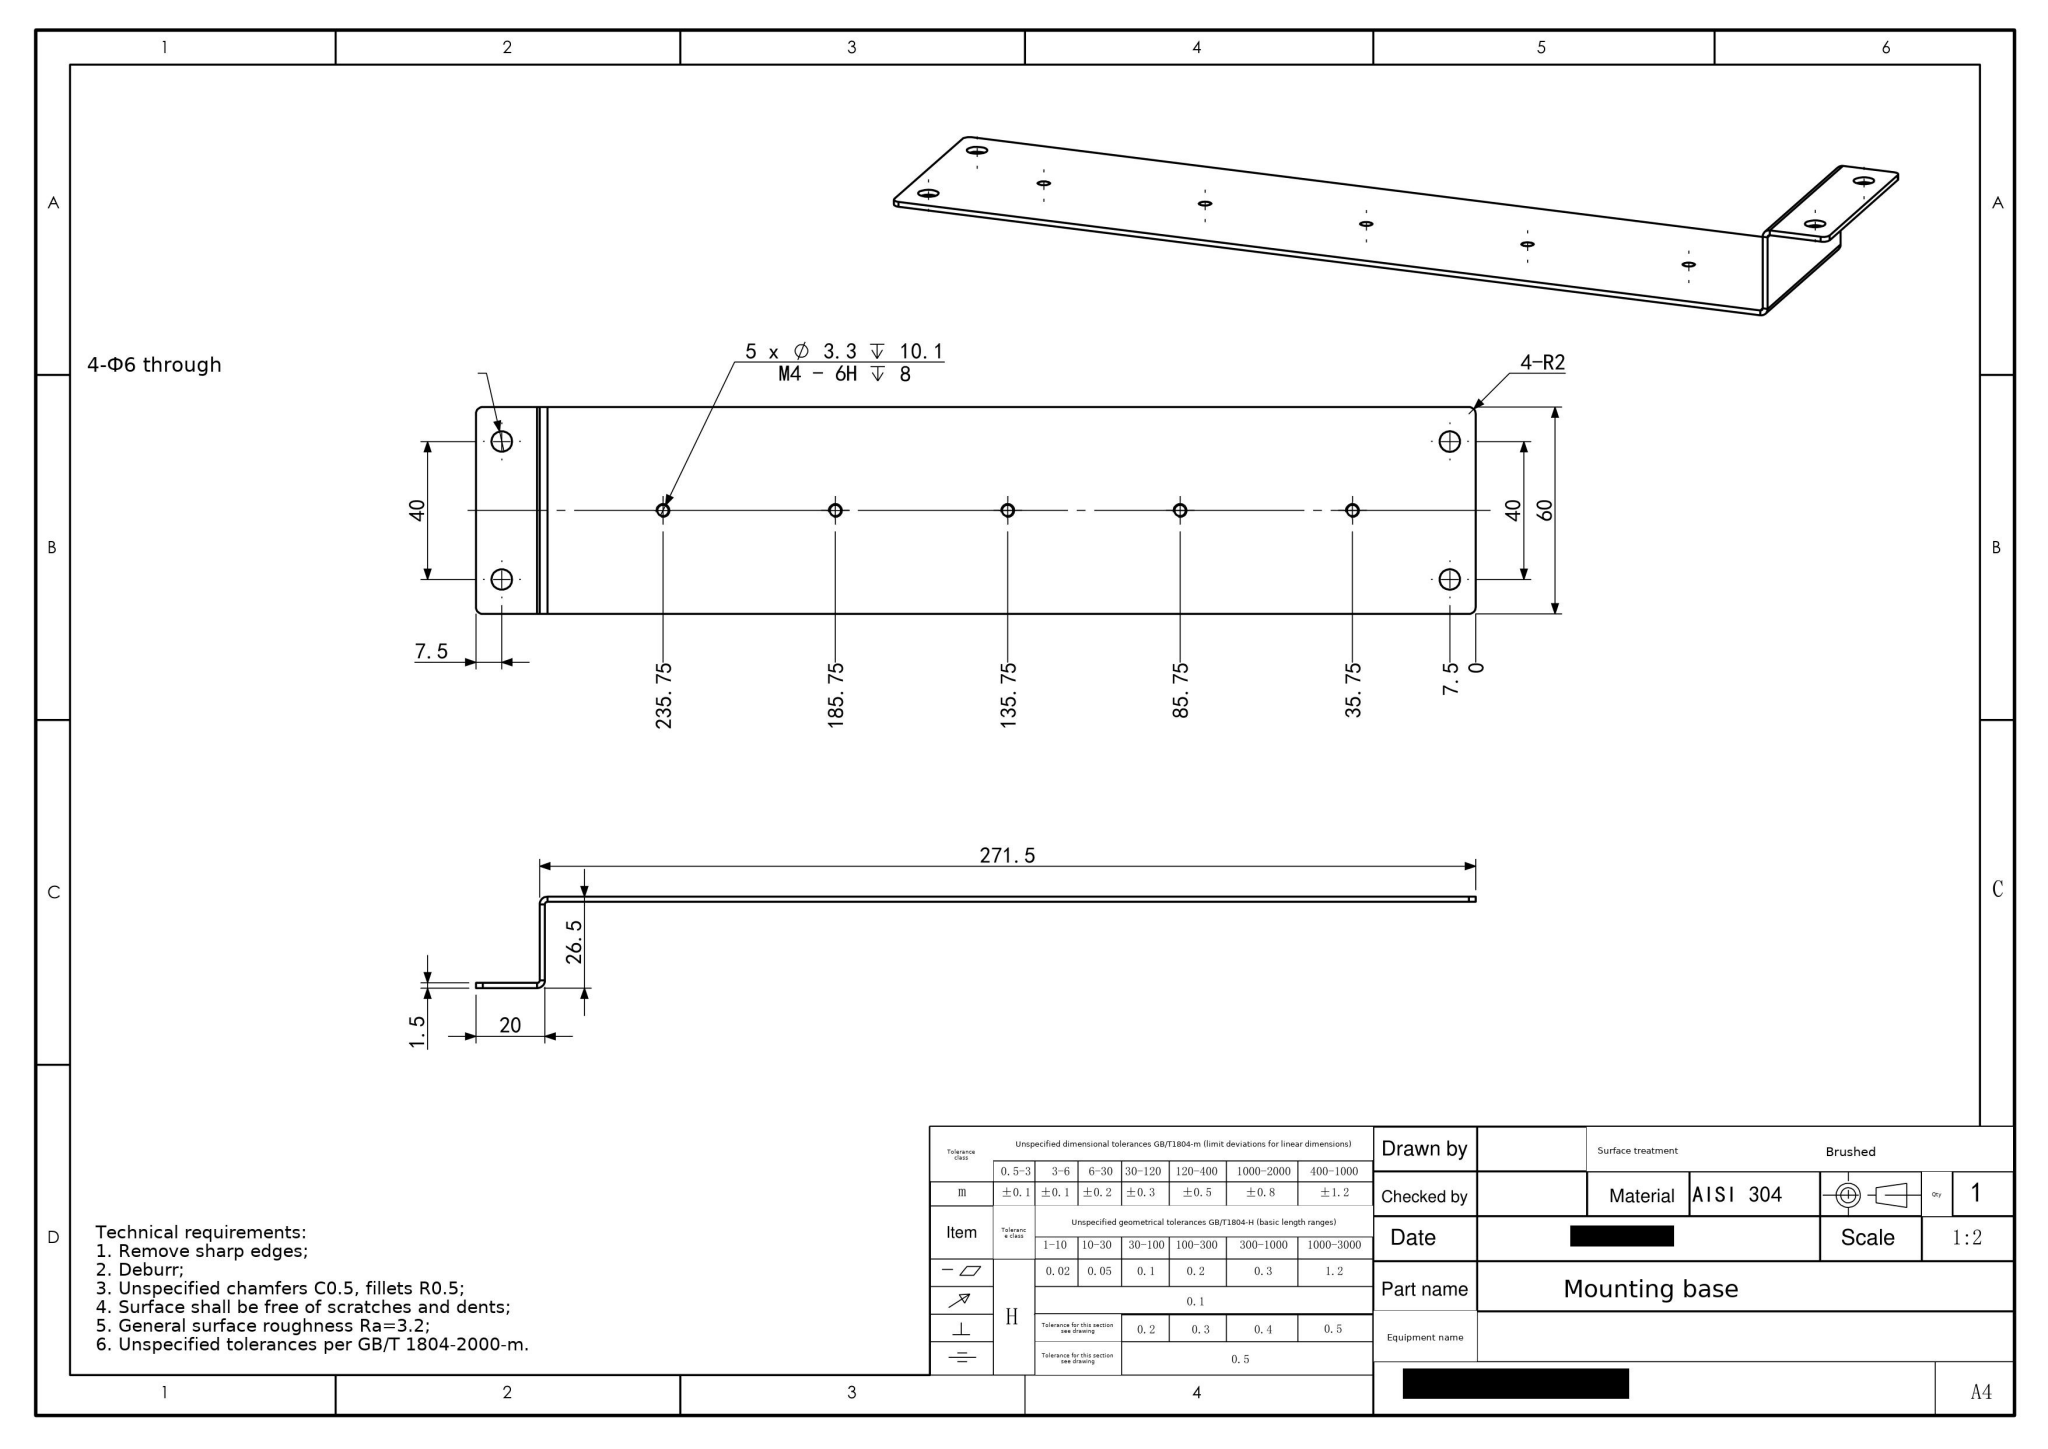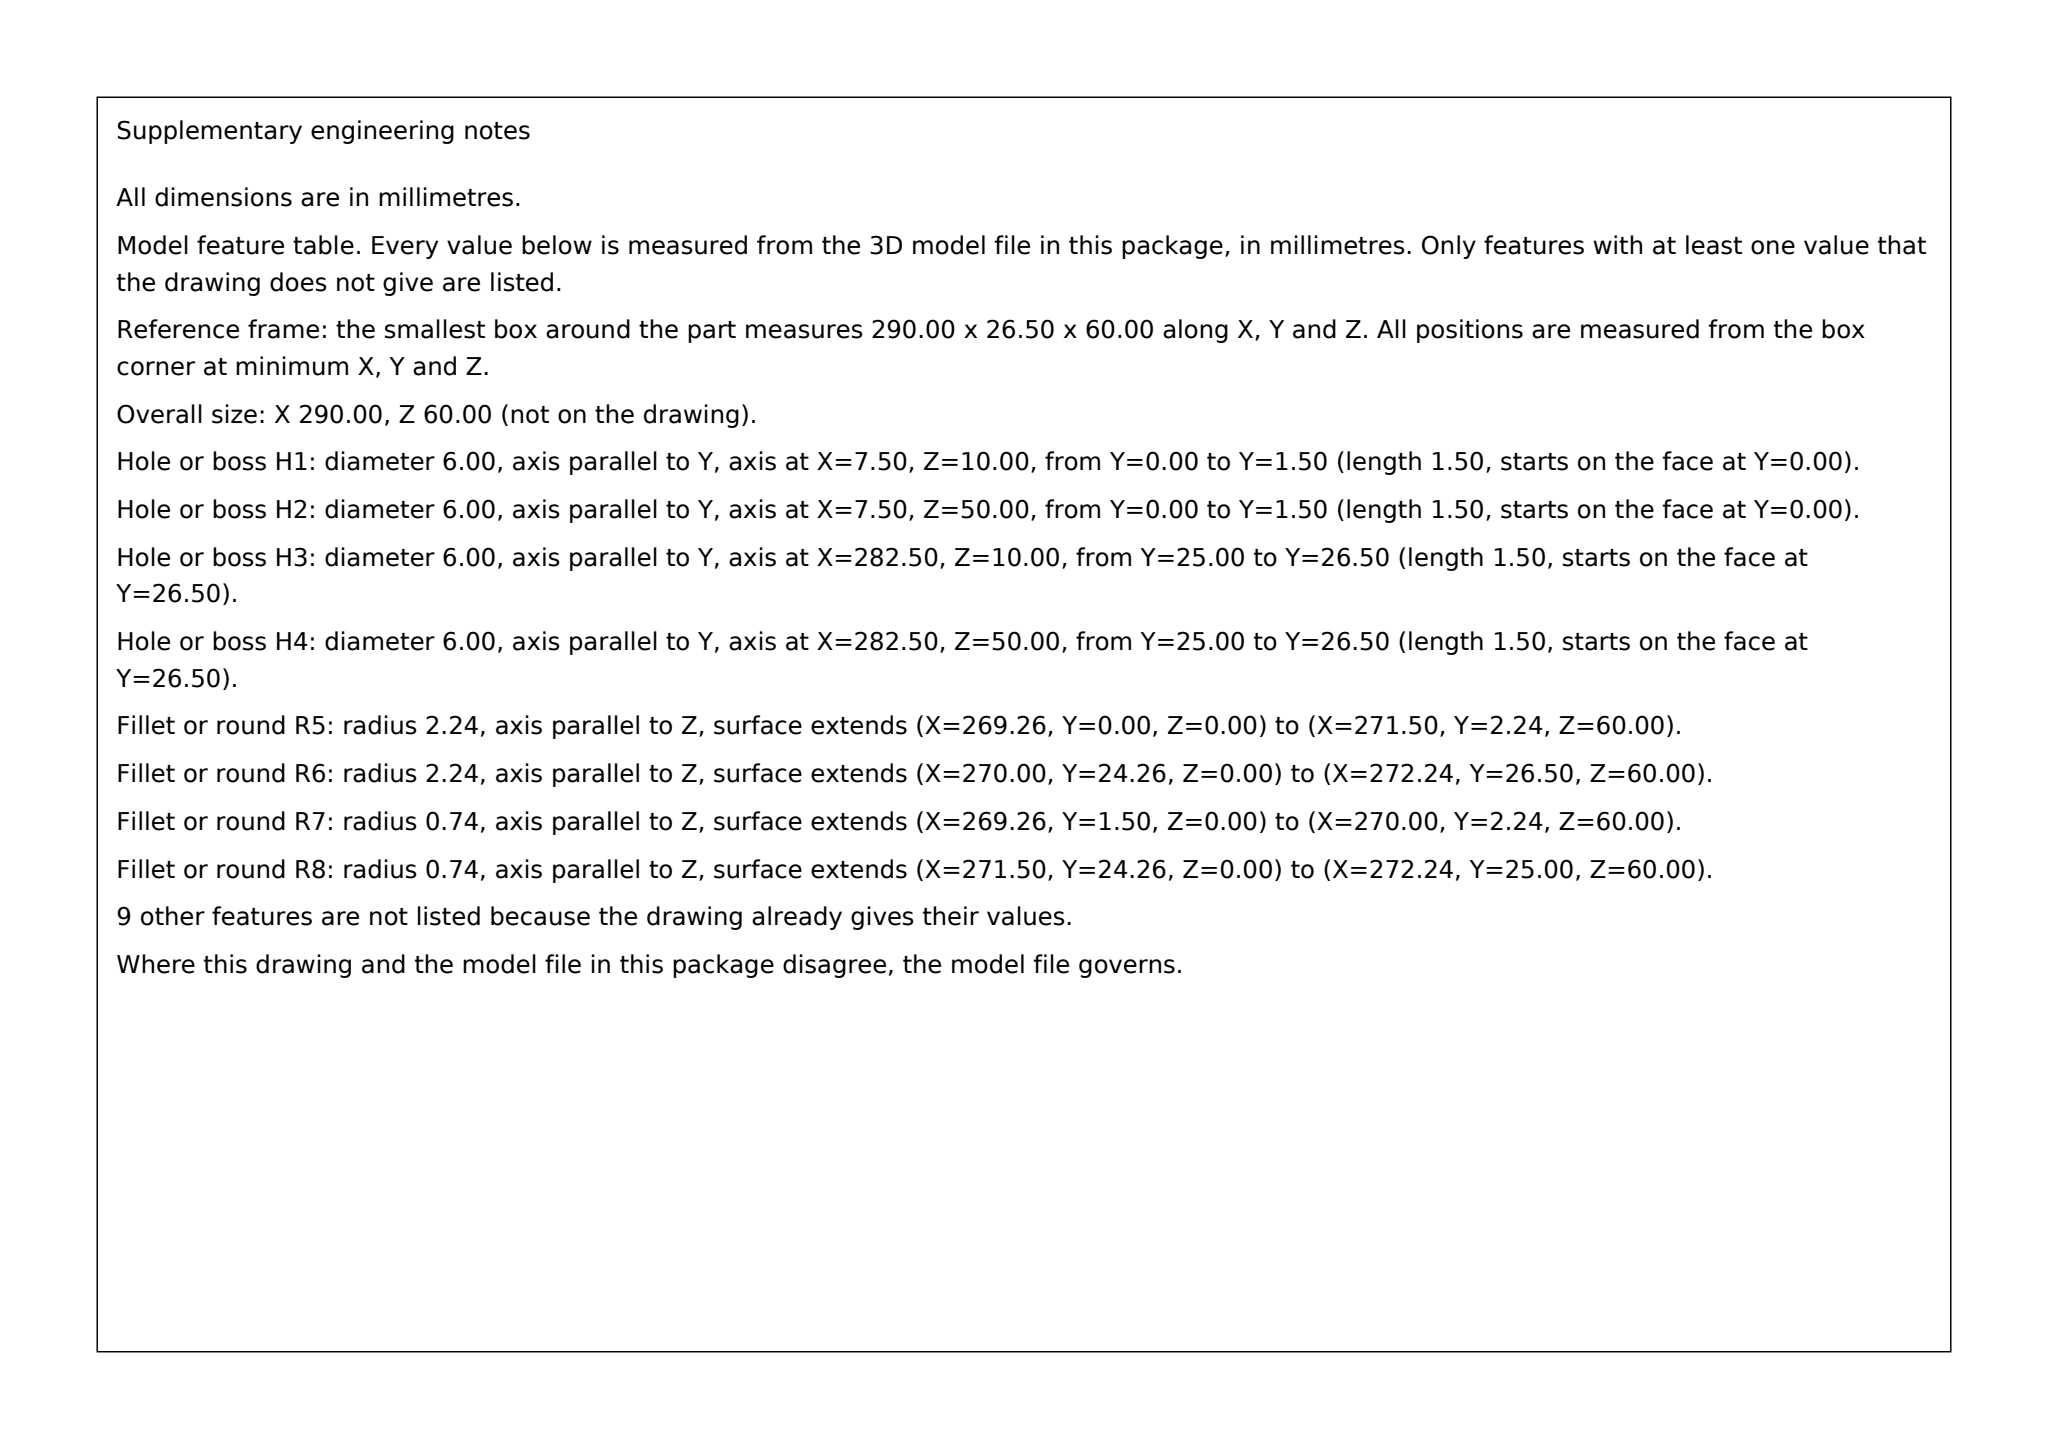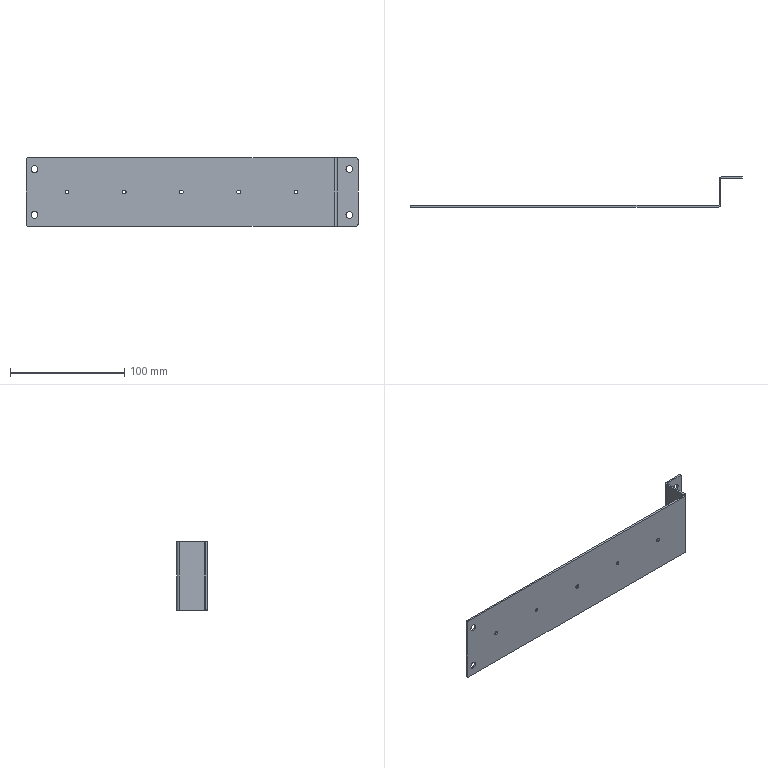Part | SolidWorks | mm | material AISI 304 | 1 solid | 44 faces | box 290 x 26.5 x 60 mm | volume 27996 mm3 | cylinder 26 | plane 18 | commonest cylinder face diameters 3.3 x10 6 x8 4 x4 4.473 x2 1.473 x2